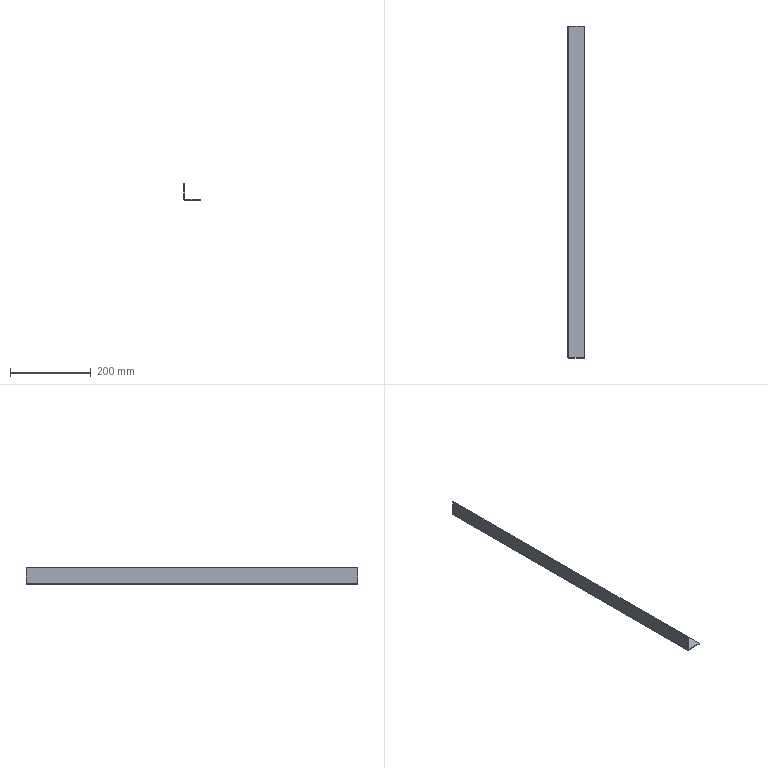Component | SolidWorks | BaseBracketAssembly-1_BaseBracketHeight-1 | 1 solid | 14 faces | box 40 x 820 x 40 mm | volume 126864 mm3 | plane 12 | cylinder 2 | commonest cylinder face diameters 5 x1 1 x1 | material 2.0mm Cold Rolled Plate
STEP:
#1=CARTESIAN_POINT('',(-13.459,-17.722,24.7));
#2=VERTEX_POINT('',#1);
#3=CARTESIAN_POINT('',(-13.459,-17.722,24.779));
#4=VERTEX_POINT('',#3);
#5=CARTESIAN_POINT('',(-13.459,-17.722,24.7));
#6=DIRECTION('',(0.,0.,1.));
#7=VECTOR('',#6,39.37);
#8=LINE('',#5,#7);
#9=EDGE_CURVE('',#2,#4,#8,.T.);
#10=ORIENTED_EDGE('',*,*,#9,.F.);
#11=CARTESIAN_POINT('',(-13.557,-17.722,24.799));
#12=VERTEX_POINT('',#11);
#13=CARTESIAN_POINT('',(-13.459,-17.722,24.799));
#14=DIRECTION('',(0.,-1.,0.));
#15=DIRECTION('',(0.,0.,1.));
#16=AXIS2_PLACEMENT_3D('',#13,#14,#15);
#17=CIRCLE('',#16,0.09843);
#18=EDGE_CURVE('',#12,#2,#17,.T.);
#19=ORIENTED_EDGE('',*,*,#18,.F.);
#20=CARTESIAN_POINT('',(-13.479,-17.722,24.799));
#21=VERTEX_POINT('',#20);
#22=CARTESIAN_POINT('',(-13.479,-17.722,24.799));
#23=DIRECTION('',(-1.,-0.,0.));
#24=VECTOR('',#23,39.37);
#25=LINE('',#22,#24);
#26=EDGE_CURVE('',#21,#12,#25,.T.);
#27=ORIENTED_EDGE('',*,*,#26,.F.);
#28=CARTESIAN_POINT('',(-13.459,-17.722,24.799));
#29=DIRECTION('',(0.,-1.,0.));
#30=DIRECTION('',(0.,0.,1.));
#31=AXIS2_PLACEMENT_3D('',#28,#29,#30);
#32=CIRCLE('',#31,0.01969);
#33=EDGE_CURVE('',#21,#4,#32,.T.);
#34=ORIENTED_EDGE('',*,*,#33,.T.);
#35=EDGE_LOOP('',(#10,#19,#27,#34));
#36=FACE_OUTER_BOUND('',#35,.T.);
#37=CARTESIAN_POINT('',(-13.459,-17.722,24.7));
#38=DIRECTION('',(-0.,1.,-0.));
#39=DIRECTION('',(0.,0.,1.));
#40=AXIS2_PLACEMENT_3D('',#37,#38,#39);
#41=PLANE('',#40);
#42=ADVANCED_FACE('',(#36),#41,.T.);
#43=CARTESIAN_POINT('',(-11.983,-17.722,24.7));
#44=VERTEX_POINT('',#43);
#45=CARTESIAN_POINT('',(-11.983,-17.722,24.7));
#46=DIRECTION('',(1.,0.,-0.));
#47=VECTOR('',#46,39.37);
#48=LINE('',#45,#47);
#49=EDGE_CURVE('',#2,#44,#48,.T.);
#50=ORIENTED_EDGE('',*,*,#49,.F.);
#51=ORIENTED_EDGE('',*,*,#9,.T.);
#52=CARTESIAN_POINT('',(-11.983,-17.722,24.779));
#53=VERTEX_POINT('',#52);
#54=CARTESIAN_POINT('',(-11.983,-17.722,24.779));
#55=DIRECTION('',(1.,0.,-0.));
#56=VECTOR('',#55,39.37);
#57=LINE('',#54,#56);
#58=EDGE_CURVE('',#4,#53,#57,.T.);
#59=ORIENTED_EDGE('',*,*,#58,.T.);
#60=CARTESIAN_POINT('',(-11.983,-17.722,24.7));
#61=DIRECTION('',(0.,0.,1.));
#62=VECTOR('',#61,39.37);
#63=LINE('',#60,#62);
#64=EDGE_CURVE('',#44,#53,#63,.T.);
#65=ORIENTED_EDGE('',*,*,#64,.F.);
#66=EDGE_LOOP('',(#50,#51,#59,#65));
#67=FACE_OUTER_BOUND('',#66,.T.);
#68=CARTESIAN_POINT('',(-13.479,-17.722,24.799));
#69=DIRECTION('',(-0.,1.,-0.));
#70=DIRECTION('',(0.,0.,1.));
#71=AXIS2_PLACEMENT_3D('',#68,#69,#70);
#72=PLANE('',#71);
#73=ADVANCED_FACE('',(#67),#72,.T.);
#74=CARTESIAN_POINT('',(-13.557,-50.005,24.799));
#75=VERTEX_POINT('',#74);
#76=CARTESIAN_POINT('',(-13.479,-50.005,24.799));
#77=VERTEX_POINT('',#76);
#78=CARTESIAN_POINT('',(-13.557,-50.005,24.799));
#79=DIRECTION('',(1.,0.,-0.));
#80=VECTOR('',#79,39.37);
#81=LINE('',#78,#80);
#82=EDGE_CURVE('',#75,#77,#81,.T.);
#83=ORIENTED_EDGE('',*,*,#82,.F.);
#84=CARTESIAN_POINT('',(-13.459,-50.005,24.7));
#85=VERTEX_POINT('',#84);
#86=CARTESIAN_POINT('',(-13.459,-50.005,24.799));
#87=DIRECTION('',(0.,-1.,0.));
#88=DIRECTION('',(0.,0.,1.));
#89=AXIS2_PLACEMENT_3D('',#86,#87,#88);
#90=CIRCLE('',#89,0.09843);
#91=EDGE_CURVE('',#75,#85,#90,.T.);
#92=ORIENTED_EDGE('',*,*,#91,.T.);
#93=CARTESIAN_POINT('',(-13.459,-50.005,24.779));
#94=VERTEX_POINT('',#93);
#95=CARTESIAN_POINT('',(-13.459,-50.005,24.779));
#96=DIRECTION('',(-0.,-0.,-1.));
#97=VECTOR('',#96,39.37);
#98=LINE('',#95,#97);
#99=EDGE_CURVE('',#94,#85,#98,.T.);
#100=ORIENTED_EDGE('',*,*,#99,.F.);
#101=CARTESIAN_POINT('',(-13.459,-50.005,24.799));
#102=DIRECTION('',(0.,-1.,0.));
#103=DIRECTION('',(0.,0.,1.));
#104=AXIS2_PLACEMENT_3D('',#101,#102,#103);
#105=CIRCLE('',#104,0.01969);
#106=EDGE_CURVE('',#77,#94,#105,.T.);
#107=ORIENTED_EDGE('',*,*,#106,.F.);
#108=EDGE_LOOP('',(#83,#92,#100,#107));
#109=FACE_OUTER_BOUND('',#108,.T.);
#110=CARTESIAN_POINT('',(-13.557,-50.005,24.799));
#111=DIRECTION('',(0.,-1.,0.));
#112=DIRECTION('',(-0.,-0.,-1.));
#113=AXIS2_PLACEMENT_3D('',#110,#111,#112);
#114=PLANE('',#113);
#115=ADVANCED_FACE('',(#109),#114,.T.);
#116=CARTESIAN_POINT('',(-13.557,-50.005,26.275));
#117=VERTEX_POINT('',#116);
#118=CARTESIAN_POINT('',(-13.557,-50.005,24.7));
#119=DIRECTION('',(-0.,-0.,-1.));
#120=VECTOR('',#119,39.37);
#121=LINE('',#118,#120);
#122=EDGE_CURVE('',#117,#75,#121,.T.);
#123=ORIENTED_EDGE('',*,*,#122,.T.);
#124=ORIENTED_EDGE('',*,*,#82,.T.);
#125=CARTESIAN_POINT('',(-13.479,-50.005,26.275));
#126=VERTEX_POINT('',#125);
#127=CARTESIAN_POINT('',(-13.479,-50.005,24.7));
#128=DIRECTION('',(-0.,-0.,-1.));
#129=VECTOR('',#128,39.37);
#130=LINE('',#127,#129);
#131=EDGE_CURVE('',#126,#77,#130,.T.);
#132=ORIENTED_EDGE('',*,*,#131,.F.);
#133=CARTESIAN_POINT('',(-13.479,-50.005,26.275));
#134=DIRECTION('',(-1.,-0.,0.));
#135=VECTOR('',#134,39.37);
#136=LINE('',#133,#135);
#137=EDGE_CURVE('',#126,#117,#136,.T.);
#138=ORIENTED_EDGE('',*,*,#137,.T.);
#139=EDGE_LOOP('',(#123,#124,#132,#138));
#140=FACE_OUTER_BOUND('',#139,.T.);
#141=CARTESIAN_POINT('',(-13.459,-50.005,24.779));
#142=DIRECTION('',(0.,-1.,0.));
#143=DIRECTION('',(-0.,-0.,-1.));
#144=AXIS2_PLACEMENT_3D('',#141,#142,#143);
#145=PLANE('',#144);
#146=ADVANCED_FACE('',(#140),#145,.T.);
#147=CARTESIAN_POINT('',(-11.983,-50.005,24.779));
#148=VERTEX_POINT('',#147);
#149=CARTESIAN_POINT('',(-11.983,-50.005,24.779));
#150=DIRECTION('',(1.,0.,-0.));
#151=VECTOR('',#150,39.37);
#152=LINE('',#149,#151);
#153=EDGE_CURVE('',#94,#148,#152,.T.);
#154=ORIENTED_EDGE('',*,*,#153,.T.);
#155=CARTESIAN_POINT('',(-11.983,-17.722,24.779));
#156=DIRECTION('',(0.,-1.,0.));
#157=VECTOR('',#156,39.37);
#158=LINE('',#155,#157);
#159=EDGE_CURVE('',#53,#148,#158,.T.);
#160=ORIENTED_EDGE('',*,*,#159,.F.);
#161=ORIENTED_EDGE('',*,*,#58,.F.);
#162=CARTESIAN_POINT('',(-13.459,-17.722,24.779));
#163=DIRECTION('',(0.,-1.,0.));
#164=VECTOR('',#163,39.37);
#165=LINE('',#162,#164);
#166=EDGE_CURVE('',#4,#94,#165,.T.);
#167=ORIENTED_EDGE('',*,*,#166,.T.);
#168=EDGE_LOOP('',(#154,#160,#161,#167));
#169=FACE_OUTER_BOUND('',#168,.T.);
#170=CARTESIAN_POINT('',(-11.983,-17.722,24.779));
#171=DIRECTION('',(-0.,-0.,-1.));
#172=DIRECTION('',(-1.,-0.,0.));
#173=AXIS2_PLACEMENT_3D('',#170,#171,#172);
#174=PLANE('',#173);
#175=ADVANCED_FACE('',(#169),#174,.F.);
#176=CARTESIAN_POINT('',(-11.983,-50.005,24.7));
#177=VERTEX_POINT('',#176);
#178=CARTESIAN_POINT('',(-11.983,-50.005,24.7));
#179=DIRECTION('',(0.,0.,1.));
#180=VECTOR('',#179,39.37);
#181=LINE('',#178,#180);
#182=EDGE_CURVE('',#177,#148,#181,.T.);
#183=ORIENTED_EDGE('',*,*,#182,.F.);
#184=CARTESIAN_POINT('',(-11.983,-17.722,24.7));
#185=DIRECTION('',(0.,-1.,0.));
#186=VECTOR('',#185,39.37);
#187=LINE('',#184,#186);
#188=EDGE_CURVE('',#44,#177,#187,.T.);
#189=ORIENTED_EDGE('',*,*,#188,.F.);
#190=ORIENTED_EDGE('',*,*,#64,.T.);
#191=ORIENTED_EDGE('',*,*,#159,.T.);
#192=EDGE_LOOP('',(#183,#189,#190,#191));
#193=FACE_OUTER_BOUND('',#192,.T.);
#194=CARTESIAN_POINT('',(-11.983,-17.722,24.7));
#195=DIRECTION('',(1.,0.,-0.));
#196=DIRECTION('',(-0.,1.,-0.));
#197=AXIS2_PLACEMENT_3D('',#194,#195,#196);
#198=PLANE('',#197);
#199=ADVANCED_FACE('',(#193),#198,.T.);
#200=CARTESIAN_POINT('',(-11.983,-50.005,24.7));
#201=DIRECTION('',(1.,0.,-0.));
#202=VECTOR('',#201,39.37);
#203=LINE('',#200,#202);
#204=EDGE_CURVE('',#85,#177,#203,.T.);
#205=ORIENTED_EDGE('',*,*,#204,.F.);
#206=CARTESIAN_POINT('',(-13.459,-17.722,24.7));
#207=DIRECTION('',(0.,-1.,0.));
#208=VECTOR('',#207,39.37);
#209=LINE('',#206,#208);
#210=EDGE_CURVE('',#2,#85,#209,.T.);
#211=ORIENTED_EDGE('',*,*,#210,.F.);
#212=ORIENTED_EDGE('',*,*,#49,.T.);
#213=ORIENTED_EDGE('',*,*,#188,.T.);
#214=EDGE_LOOP('',(#205,#211,#212,#213));
#215=FACE_OUTER_BOUND('',#214,.T.);
#216=CARTESIAN_POINT('',(-11.983,-17.722,24.7));
#217=DIRECTION('',(-0.,-0.,-1.));
#218=DIRECTION('',(-1.,-0.,0.));
#219=AXIS2_PLACEMENT_3D('',#216,#217,#218);
#220=PLANE('',#219);
#221=ADVANCED_FACE('',(#215),#220,.T.);
#222=ORIENTED_EDGE('',*,*,#91,.F.);
#223=CARTESIAN_POINT('',(-13.557,-17.722,24.799));
#224=DIRECTION('',(0.,-1.,0.));
#225=VECTOR('',#224,39.37);
#226=LINE('',#223,#225);
#227=EDGE_CURVE('',#12,#75,#226,.T.);
#228=ORIENTED_EDGE('',*,*,#227,.F.);
#229=ORIENTED_EDGE('',*,*,#18,.T.);
#230=ORIENTED_EDGE('',*,*,#210,.T.);
#231=EDGE_LOOP('',(#222,#228,#229,#230));
#232=FACE_OUTER_BOUND('',#231,.T.);
#233=CARTESIAN_POINT('',(-13.459,-17.722,24.799));
#234=DIRECTION('',(0.,-1.,0.));
#235=DIRECTION('',(0.,0.,-1.));
#236=AXIS2_PLACEMENT_3D('',#233,#234,#235);
#237=CYLINDRICAL_SURFACE('',#236,0.09843);
#238=ADVANCED_FACE('',(#232),#237,.T.);
#239=ORIENTED_EDGE('',*,*,#122,.F.);
#240=CARTESIAN_POINT('',(-13.557,-17.722,26.275));
#241=VERTEX_POINT('',#240);
#242=CARTESIAN_POINT('',(-13.557,-17.722,26.275));
#243=DIRECTION('',(0.,-1.,0.));
#244=VECTOR('',#243,39.37);
#245=LINE('',#242,#244);
#246=EDGE_CURVE('',#241,#117,#245,.T.);
#247=ORIENTED_EDGE('',*,*,#246,.F.);
#248=CARTESIAN_POINT('',(-13.557,-17.722,24.7));
#249=DIRECTION('',(-0.,-0.,-1.));
#250=VECTOR('',#249,39.37);
#251=LINE('',#248,#250);
#252=EDGE_CURVE('',#241,#12,#251,.T.);
#253=ORIENTED_EDGE('',*,*,#252,.T.);
#254=ORIENTED_EDGE('',*,*,#227,.T.);
#255=EDGE_LOOP('',(#239,#247,#253,#254));
#256=FACE_OUTER_BOUND('',#255,.T.);
#257=CARTESIAN_POINT('',(-13.557,-17.722,24.7));
#258=DIRECTION('',(-1.,-0.,0.));
#259=DIRECTION('',(0.,-1.,0.));
#260=AXIS2_PLACEMENT_3D('',#257,#258,#259);
#261=PLANE('',#260);
#262=ADVANCED_FACE('',(#256),#261,.T.);
#263=ORIENTED_EDGE('',*,*,#137,.F.);
#264=CARTESIAN_POINT('',(-13.479,-17.722,26.275));
#265=VERTEX_POINT('',#264);
#266=CARTESIAN_POINT('',(-13.479,-17.722,26.275));
#267=DIRECTION('',(0.,-1.,0.));
#268=VECTOR('',#267,39.37);
#269=LINE('',#266,#268);
#270=EDGE_CURVE('',#265,#126,#269,.T.);
#271=ORIENTED_EDGE('',*,*,#270,.F.);
#272=CARTESIAN_POINT('',(-13.479,-17.722,26.275));
#273=DIRECTION('',(-1.,-0.,0.));
#274=VECTOR('',#273,39.37);
#275=LINE('',#272,#274);
#276=EDGE_CURVE('',#265,#241,#275,.T.);
#277=ORIENTED_EDGE('',*,*,#276,.T.);
#278=ORIENTED_EDGE('',*,*,#246,.T.);
#279=EDGE_LOOP('',(#263,#271,#277,#278));
#280=FACE_OUTER_BOUND('',#279,.T.);
#281=CARTESIAN_POINT('',(-13.479,-17.722,26.275));
#282=DIRECTION('',(0.,0.,1.));
#283=DIRECTION('',(0.,-1.,0.));
#284=AXIS2_PLACEMENT_3D('',#281,#282,#283);
#285=PLANE('',#284);
#286=ADVANCED_FACE('',(#280),#285,.T.);
#287=ORIENTED_EDGE('',*,*,#131,.T.);
#288=CARTESIAN_POINT('',(-13.479,-17.722,24.799));
#289=DIRECTION('',(0.,-1.,0.));
#290=VECTOR('',#289,39.37);
#291=LINE('',#288,#290);
#292=EDGE_CURVE('',#21,#77,#291,.T.);
#293=ORIENTED_EDGE('',*,*,#292,.F.);
#294=CARTESIAN_POINT('',(-13.479,-17.722,24.7));
#295=DIRECTION('',(-0.,-0.,-1.));
#296=VECTOR('',#295,39.37);
#297=LINE('',#294,#296);
#298=EDGE_CURVE('',#265,#21,#297,.T.);
#299=ORIENTED_EDGE('',*,*,#298,.F.);
#300=ORIENTED_EDGE('',*,*,#270,.T.);
#301=EDGE_LOOP('',(#287,#293,#299,#300));
#302=FACE_OUTER_BOUND('',#301,.T.);
#303=CARTESIAN_POINT('',(-13.479,-17.722,24.7));
#304=DIRECTION('',(-1.,-0.,0.));
#305=DIRECTION('',(0.,-1.,0.));
#306=AXIS2_PLACEMENT_3D('',#303,#304,#305);
#307=PLANE('',#306);
#308=ADVANCED_FACE('',(#302),#307,.F.);
#309=ORIENTED_EDGE('',*,*,#106,.T.);
#310=ORIENTED_EDGE('',*,*,#166,.F.);
#311=ORIENTED_EDGE('',*,*,#33,.F.);
#312=ORIENTED_EDGE('',*,*,#292,.T.);
#313=EDGE_LOOP('',(#309,#310,#311,#312));
#314=FACE_OUTER_BOUND('',#313,.T.);
#315=CARTESIAN_POINT('',(-13.459,-17.722,24.799));
#316=DIRECTION('',(0.,-1.,0.));
#317=DIRECTION('',(0.,0.,-1.));
#318=AXIS2_PLACEMENT_3D('',#315,#316,#317);
#319=CYLINDRICAL_SURFACE('',#318,0.01969);
#320=ADVANCED_FACE('',(#314),#319,.F.);
#321=ORIENTED_EDGE('',*,*,#298,.T.);
#322=ORIENTED_EDGE('',*,*,#26,.T.);
#323=ORIENTED_EDGE('',*,*,#252,.F.);
#324=ORIENTED_EDGE('',*,*,#276,.F.);
#325=EDGE_LOOP('',(#321,#322,#323,#324));
#326=FACE_OUTER_BOUND('',#325,.T.);
#327=CARTESIAN_POINT('',(-13.459,-17.722,24.799));
#328=DIRECTION('',(-0.,1.,-0.));
#329=DIRECTION('',(0.,0.,1.));
#330=AXIS2_PLACEMENT_3D('',#327,#328,#329);
#331=PLANE('',#330);
#332=ADVANCED_FACE('',(#326),#331,.T.);
#333=ORIENTED_EDGE('',*,*,#153,.F.);
#334=ORIENTED_EDGE('',*,*,#99,.T.);
#335=ORIENTED_EDGE('',*,*,#204,.T.);
#336=ORIENTED_EDGE('',*,*,#182,.T.);
#337=EDGE_LOOP('',(#333,#334,#335,#336));
#338=FACE_OUTER_BOUND('',#337,.T.);
#339=CARTESIAN_POINT('',(-13.459,-50.005,24.799));
#340=DIRECTION('',(-0.,1.,-0.));
#341=DIRECTION('',(0.,0.,1.));
#342=AXIS2_PLACEMENT_3D('',#339,#340,#341);
#343=PLANE('',#342);
#344=ADVANCED_FACE('',(#338),#343,.F.);
#345=CLOSED_SHELL('',(#42,#73,#115,#146,#175,#199,#221,#238,#262,#286,#308,#320,#332,#344));
#346=MANIFOLD_SOLID_BREP('',#345);
#347=CARTESIAN_POINT('',(0.,0.,0.));
#348=DIRECTION('',(0.,0.,1.));
#349=DIRECTION('',(1.,0.,0.));
#350=AXIS2_PLACEMENT_3D('',#347,#348,#349);
#351=(LENGTH_UNIT()NAMED_UNIT(*)SI_UNIT($,.METRE.));
#352=LENGTH_MEASURE_WITH_UNIT(LENGTH_MEASURE(0.0254),#351);
#353=DIMENSIONAL_EXPONENTS(1.,0.,0.,0.,0.,0.,0.);
#354=(CONVERSION_BASED_UNIT('',#352)LENGTH_UNIT()NAMED_UNIT(#353));
#355=UNCERTAINTY_MEASURE_WITH_UNIT(LENGTH_MEASURE(0.00001),#354,'','');
#356=(NAMED_UNIT(*)PLANE_ANGLE_UNIT()SI_UNIT($,.RADIAN.));
#357=(NAMED_UNIT(*)SI_UNIT($,.STERADIAN.)SOLID_ANGLE_UNIT());
#358=(GEOMETRIC_REPRESENTATION_CONTEXT(3)GLOBAL_UNCERTAINTY_ASSIGNED_CONTEXT((#355))GLOBAL_UNIT_ASSIGNED_CONTEXT((#354,#356,#357))REPRESENTATION_CONTEXT('',''));
#359=ADVANCED_BREP_SHAPE_REPRESENTATION('',(#346,#350),#358);
#360=COLOUR_RGB('',0.7922,0.8196,0.9333);
#361=FILL_AREA_STYLE_COLOUR('',#360);
#362=FILL_AREA_STYLE('',(#361));
#363=SURFACE_STYLE_FILL_AREA(#362);
#364=SURFACE_SIDE_STYLE('',(#363));
#365=SURFACE_STYLE_USAGE(.BOTH.,#364);
#366=PRESENTATION_STYLE_ASSIGNMENT((#365));
#367=STYLED_ITEM('',(#366),#346);
#368=(LENGTH_UNIT()NAMED_UNIT(*)SI_UNIT($,.METRE.));
#369=LENGTH_MEASURE_WITH_UNIT(LENGTH_MEASURE(0.0254),#368);
#370=DIMENSIONAL_EXPONENTS(1.,0.,0.,0.,0.,0.,0.);
#371=(CONVERSION_BASED_UNIT('',#369)LENGTH_UNIT()NAMED_UNIT(#370));
#372=UNCERTAINTY_MEASURE_WITH_UNIT(LENGTH_MEASURE(0.00001),#371,'','');
#373=(NAMED_UNIT(*)PLANE_ANGLE_UNIT()SI_UNIT($,.RADIAN.));
#374=(NAMED_UNIT(*)SI_UNIT($,.STERADIAN.)SOLID_ANGLE_UNIT());
#375=(GEOMETRIC_REPRESENTATION_CONTEXT(3)GLOBAL_UNCERTAINTY_ASSIGNED_CONTEXT((#372))GLOBAL_UNIT_ASSIGNED_CONTEXT((#371,#373,#374))REPRESENTATION_CONTEXT('',''));
#376=MECHANICAL_DESIGN_GEOMETRIC_PRESENTATION_REPRESENTATION('',(#367),#375);
#377=PRESENTATION_LAYER_ASSIGNMENT('','',(#367));